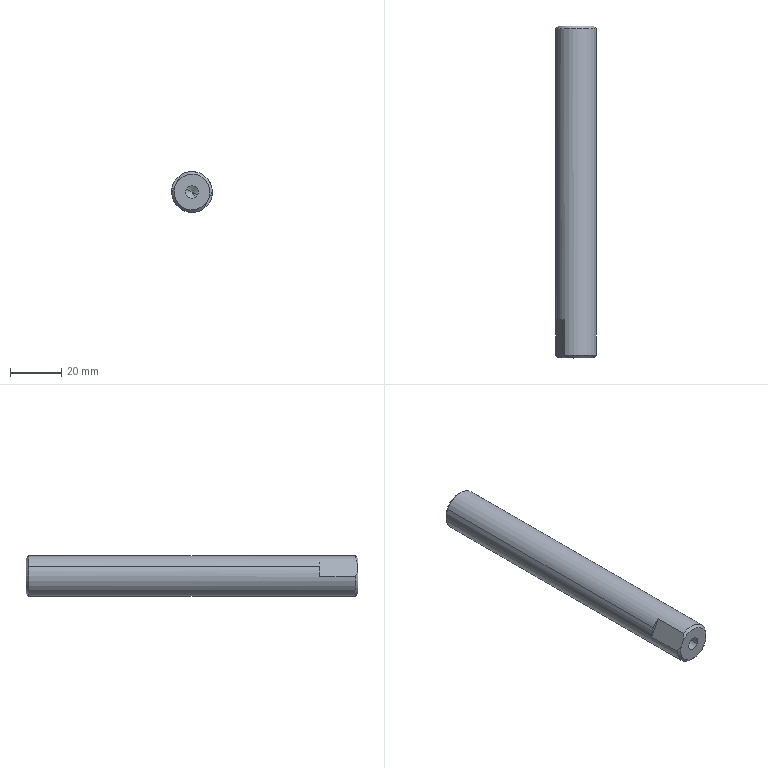Component | SolidWorks | PressingMechanism-25-2 | 1 solid | 16 faces | box 16 x 130 x 16 mm | volume 25596 mm3 | cone 6 | plane 6 | cylinder 4 | commonest cylinder face diameters 5 x2 16 x2
build123d program:
from build123d import *

# Parameters (mm, degrees)
SKETCH1_R             = 8
EXTRUDE1_DEPTH        = 130
M6_TAPPED_HOLE1_D     = 5
M6_TAPPED_HOLE1_DEPTH = 17
M6_TAPPED_HOLE1_TIP   = 1.502
CHAMFER1_SIZE         = 1
EXTRUDE2_DEPTH        = 131.491
EXTRUDE2_DEPTH_BACK   = 131.491
SKETCH4_W             = 15
SKETCH4_H             = 1


with BuildPart() as part:
    # Sketch1 → Extrude1 (new body)
    with BuildSketch(Plane(origin=(0, 0, 0), x_dir=(0, 0, -1), z_dir=(1, 0, 0))):
        Circle(SKETCH1_R)
    extrude(amount=EXTRUDE1_DEPTH)

    # M6 Tapped Hole1
    with Locations(Plane(origin=(130, 0, 0), x_dir=(0, 0, -1), z_dir=(1, 0, 0))):
        with Locations((0, 0)):
            Hole(M6_TAPPED_HOLE1_D / 2, depth=M6_TAPPED_HOLE1_DEPTH)
            with Locations((0, 0, -(M6_TAPPED_HOLE1_DEPTH + M6_TAPPED_HOLE1_TIP / 2))):  # 118° drill point
                Cone(0, M6_TAPPED_HOLE1_D / 2, M6_TAPPED_HOLE1_TIP, mode=Mode.SUBTRACT)

    # Chamfer1
    chamfer1_edges = [part.edges().sort_by_distance(p)[0] for p in [
        (0, 0, 8),
        (130, 0, 8),
    ]]
    chamfer(chamfer1_edges, length=CHAMFER1_SIZE)

    # Sketch4 → Extrude2 (cut, two sides: drawn at the far end of the back side and taken through both)
    with BuildSketch(Plane(origin=(0, 0, 0), x_dir=(1, 0, 0), z_dir=(0, 1, 0)).offset(-EXTRUDE2_DEPTH_BACK)):
        with Locations((122.5, 7.5)):
            Rectangle(SKETCH4_W, SKETCH4_H)
        with Locations((122.5, -7.5)):
            Rectangle(SKETCH4_W, SKETCH4_H)
    extrude(amount=EXTRUDE2_DEPTH + EXTRUDE2_DEPTH_BACK, mode=Mode.SUBTRACT)


solid = part.part

# Placed as in the assembly
solid = solid.moved(Location((0, -129, 61), (0, -62.719, -90)))
STEP:
#1=COLOUR_RGB('',0.7922,0.8196,0.9333);
#2=FILL_AREA_STYLE_COLOUR('',#1);
#3=FILL_AREA_STYLE('',(#2));
#4=SURFACE_STYLE_FILL_AREA(#3);
#5=SURFACE_SIDE_STYLE('',(#4));
#6=SURFACE_STYLE_USAGE(.BOTH.,#5);
#7=PRESENTATION_STYLE_ASSIGNMENT((#6));
#8=CARTESIAN_POINT('',(-0.2449,-5.079,2.528));
#9=VERTEX_POINT('',#8);
#10=CARTESIAN_POINT('',(0.2449,-5.079,2.275));
#11=VERTEX_POINT('',#10);
#12=CARTESIAN_POINT('',(0.,-5.079,2.402));
#13=DIRECTION('',(0.,1.,0.));
#14=DIRECTION('',(0.8888,0.,-0.4583));
#15=AXIS2_PLACEMENT_3D('',#12,#13,#14);
#16=CIRCLE('',#15,0.2756);
#17=EDGE_CURVE('',#9,#11,#16,.T.);
#18=ORIENTED_EDGE('',*,*,#17,.F.);
#19=CARTESIAN_POINT('',(-0.2799,-5.118,2.546));
#20=VERTEX_POINT('',#19);
#21=CARTESIAN_POINT('',(-0.2799,-5.118,2.546));
#22=DIRECTION('',(-0.6285,-0.7071,0.3241));
#23=VECTOR('',#22,39.37);
#24=LINE('',#21,#23);
#25=EDGE_CURVE('',#9,#20,#24,.T.);
#26=ORIENTED_EDGE('',*,*,#25,.T.);
#27=CARTESIAN_POINT('',(0.2799,-5.118,2.257));
#28=VERTEX_POINT('',#27);
#29=CARTESIAN_POINT('',(0.,-5.118,2.402));
#30=DIRECTION('',(0.,-1.,0.));
#31=DIRECTION('',(0.8888,0.,-0.4583));
#32=AXIS2_PLACEMENT_3D('',#29,#30,#31);
#33=CIRCLE('',#32,0.315);
#34=EDGE_CURVE('',#28,#20,#33,.T.);
#35=ORIENTED_EDGE('',*,*,#34,.F.);
#36=CARTESIAN_POINT('',(0.2799,-5.118,2.257));
#37=DIRECTION('',(0.6285,-0.7071,-0.3241));
#38=VECTOR('',#37,39.37);
#39=LINE('',#36,#38);
#40=EDGE_CURVE('',#11,#28,#39,.T.);
#41=ORIENTED_EDGE('',*,*,#40,.F.);
#42=EDGE_LOOP('',(#18,#26,#35,#41));
#43=FACE_OUTER_BOUND('',#42,.T.);
#44=CARTESIAN_POINT('',(0.,-5.118,2.402));
#45=DIRECTION('',(0.,-1.,0.));
#46=DIRECTION('',(0.8888,0.,-0.4583));
#47=AXIS2_PLACEMENT_3D('',#44,#45,#46);
#48=CONICAL_SURFACE('',#47,0.315,0.7854);
#49=ADVANCED_FACE('',(#43),#48,.T.);
#50=CARTESIAN_POINT('',(-0.08748,-9.528,2.447));
#51=VERTEX_POINT('',#50);
#52=CARTESIAN_POINT('',(0.08748,-9.528,2.356));
#53=VERTEX_POINT('',#52);
#54=CARTESIAN_POINT('',(0.,-9.528,2.402));
#55=DIRECTION('',(0.,-1.,0.));
#56=DIRECTION('',(0.8888,0.,-0.4583));
#57=AXIS2_PLACEMENT_3D('',#54,#55,#56);
#58=CIRCLE('',#57,0.09843);
#59=EDGE_CURVE('',#51,#53,#58,.T.);
#60=ORIENTED_EDGE('',*,*,#59,.F.);
#61=CARTESIAN_POINT('',(-0.08748,-10.197,2.447));
#62=VERTEX_POINT('',#61);
#63=CARTESIAN_POINT('',(-0.08748,-10.197,2.447));
#64=DIRECTION('',(0.,-1.,0.));
#65=VECTOR('',#64,39.37);
#66=LINE('',#63,#65);
#67=EDGE_CURVE('',#51,#62,#66,.T.);
#68=ORIENTED_EDGE('',*,*,#67,.T.);
#69=CARTESIAN_POINT('',(0.08748,-10.197,2.356));
#70=VERTEX_POINT('',#69);
#71=CARTESIAN_POINT('',(0.,-10.197,2.402));
#72=DIRECTION('',(0.,-1.,0.));
#73=DIRECTION('',(0.8888,0.,-0.4583));
#74=AXIS2_PLACEMENT_3D('',#71,#72,#73);
#75=CIRCLE('',#74,0.09843);
#76=EDGE_CURVE('',#62,#70,#75,.T.);
#77=ORIENTED_EDGE('',*,*,#76,.T.);
#78=CARTESIAN_POINT('',(0.08748,-10.197,2.356));
#79=DIRECTION('',(0.,-1.,0.));
#80=VECTOR('',#79,39.37);
#81=LINE('',#78,#80);
#82=EDGE_CURVE('',#53,#70,#81,.T.);
#83=ORIENTED_EDGE('',*,*,#82,.F.);
#84=EDGE_LOOP('',(#60,#68,#77,#83));
#85=FACE_OUTER_BOUND('',#84,.T.);
#86=CARTESIAN_POINT('',(0.,-10.197,2.402));
#87=DIRECTION('',(0.,-1.,0.));
#88=DIRECTION('',(0.8888,0.,-0.4583));
#89=AXIS2_PLACEMENT_3D('',#86,#87,#88);
#90=CYLINDRICAL_SURFACE('',#89,0.09843);
#91=ADVANCED_FACE('',(#85),#90,.F.);
#92=CARTESIAN_POINT('',(0.,-9.468,2.402));
#93=VERTEX_POINT('',#92);
#94=CARTESIAN_POINT('',(0.08748,-9.528,2.356));
#95=DIRECTION('',(0.7618,-0.515,-0.3929));
#96=VECTOR('',#95,39.37);
#97=LINE('',#94,#96);
#98=EDGE_CURVE('',#93,#53,#97,.T.);
#99=ORIENTED_EDGE('',*,*,#98,.F.);
#100=CARTESIAN_POINT('',(-0.08748,-9.528,2.447));
#101=DIRECTION('',(-0.7618,-0.515,0.3929));
#102=VECTOR('',#101,39.37);
#103=LINE('',#100,#102);
#104=EDGE_CURVE('',#93,#51,#103,.T.);
#105=ORIENTED_EDGE('',*,*,#104,.T.);
#106=ORIENTED_EDGE('',*,*,#59,.T.);
#107=EDGE_LOOP('',(#99,#105,#106));
#108=FACE_OUTER_BOUND('',#107,.T.);
#109=CARTESIAN_POINT('',(0.,-9.528,2.402));
#110=DIRECTION('',(0.,-1.,0.));
#111=DIRECTION('',(0.8888,0.,-0.4583));
#112=AXIS2_PLACEMENT_3D('',#109,#110,#111);
#113=CONICAL_SURFACE('',#112,0.09843,1.03);
#114=ADVANCED_FACE('',(#108),#113,.F.);
#115=CARTESIAN_POINT('',(0.3148,-9.606,2.411));
#116=VERTEX_POINT('',#115);
#117=CARTESIAN_POINT('',(0.2799,-9.606,2.257));
#118=VERTEX_POINT('',#117);
#119=CARTESIAN_POINT('',(0.,-9.606,2.402));
#120=DIRECTION('',(0.,1.,0.));
#121=DIRECTION('',(-0.8888,0.,0.4583));
#122=AXIS2_PLACEMENT_3D('',#119,#120,#121);
#123=CIRCLE('',#122,0.315);
#124=EDGE_CURVE('',#116,#118,#123,.T.);
#125=ORIENTED_EDGE('',*,*,#124,.T.);
#126=CARTESIAN_POINT('',(0.2799,-10.197,2.257));
#127=DIRECTION('',(0.,1.,0.));
#128=VECTOR('',#127,39.37);
#129=LINE('',#126,#128);
#130=EDGE_CURVE('',#118,#28,#129,.T.);
#131=ORIENTED_EDGE('',*,*,#130,.T.);
#132=ORIENTED_EDGE('',*,*,#34,.T.);
#133=CARTESIAN_POINT('',(-0.2799,-9.606,2.546));
#134=VERTEX_POINT('',#133);
#135=CARTESIAN_POINT('',(-0.2799,-10.197,2.546));
#136=DIRECTION('',(0.,1.,0.));
#137=VECTOR('',#136,39.37);
#138=LINE('',#135,#137);
#139=EDGE_CURVE('',#134,#20,#138,.T.);
#140=ORIENTED_EDGE('',*,*,#139,.F.);
#141=CARTESIAN_POINT('',(-0.1751,-9.606,2.663));
#142=VERTEX_POINT('',#141);
#143=CARTESIAN_POINT('',(0.,-9.606,2.402));
#144=DIRECTION('',(0.,1.,0.));
#145=DIRECTION('',(-0.8888,0.,0.4583));
#146=AXIS2_PLACEMENT_3D('',#143,#144,#145);
#147=CIRCLE('',#146,0.315);
#148=EDGE_CURVE('',#134,#142,#147,.T.);
#149=ORIENTED_EDGE('',*,*,#148,.T.);
#150=CARTESIAN_POINT('',(-0.1751,-10.157,2.663));
#151=VERTEX_POINT('',#150);
#152=CARTESIAN_POINT('',(-0.1751,-10.197,2.663));
#153=DIRECTION('',(0.,-1.,0.));
#154=VECTOR('',#153,39.37);
#155=LINE('',#152,#154);
#156=EDGE_CURVE('',#142,#151,#155,.T.);
#157=ORIENTED_EDGE('',*,*,#156,.T.);
#158=CARTESIAN_POINT('',(0.3148,-10.157,2.411));
#159=VERTEX_POINT('',#158);
#160=CARTESIAN_POINT('',(0.,-10.157,2.402));
#161=DIRECTION('',(0.,1.,0.));
#162=DIRECTION('',(0.8888,0.,-0.4583));
#163=AXIS2_PLACEMENT_3D('',#160,#161,#162);
#164=CIRCLE('',#163,0.315);
#165=EDGE_CURVE('',#151,#159,#164,.T.);
#166=ORIENTED_EDGE('',*,*,#165,.T.);
#167=CARTESIAN_POINT('',(0.3148,-10.197,2.411));
#168=DIRECTION('',(0.,1.,0.));
#169=VECTOR('',#168,39.37);
#170=LINE('',#167,#169);
#171=EDGE_CURVE('',#159,#116,#170,.T.);
#172=ORIENTED_EDGE('',*,*,#171,.T.);
#173=EDGE_LOOP('',(#125,#131,#132,#140,#149,#157,#166,#172));
#174=FACE_OUTER_BOUND('',#173,.T.);
#175=CARTESIAN_POINT('',(0.,-10.197,2.402));
#176=DIRECTION('',(0.,1.,0.));
#177=DIRECTION('',(-0.8888,0.,0.4583));
#178=AXIS2_PLACEMENT_3D('',#175,#176,#177);
#179=CYLINDRICAL_SURFACE('',#178,0.315);
#180=ADVANCED_FACE('',(#174),#179,.T.);
#181=CARTESIAN_POINT('',(-0.3148,-10.157,2.392));
#182=VERTEX_POINT('',#181);
#183=CARTESIAN_POINT('',(-0.2449,-10.197,2.528));
#184=VERTEX_POINT('',#183);
#185=CARTESIAN_POINT('',(-0.3148,-10.157,2.392));
#186=CARTESIAN_POINT('',(-0.3041,-10.169,2.413));
#187=CARTESIAN_POINT('',(-0.2929,-10.179,2.435));
#188=CARTESIAN_POINT('',(-0.2692,-10.193,2.481));
#189=CARTESIAN_POINT('',(-0.2572,-10.197,2.504));
#190=CARTESIAN_POINT('',(-0.2449,-10.197,2.528));
#191=B_SPLINE_CURVE_WITH_KNOTS('',3,(#185,#186,#187,#188,#189,#190),.UNSPECIFIED.,.F.,.F.,(4,2,4),(0.02013,0.02213,0.02413),.UNSPECIFIED.);
#192=EDGE_CURVE('',#182,#184,#191,.T.);
#193=ORIENTED_EDGE('',*,*,#192,.F.);
#194=CARTESIAN_POINT('',(0.1751,-10.157,2.14));
#195=VERTEX_POINT('',#194);
#196=CARTESIAN_POINT('',(0.,-10.157,2.402));
#197=DIRECTION('',(0.,1.,0.));
#198=DIRECTION('',(0.8888,0.,-0.4583));
#199=AXIS2_PLACEMENT_3D('',#196,#197,#198);
#200=CIRCLE('',#199,0.315);
#201=EDGE_CURVE('',#195,#182,#200,.T.);
#202=ORIENTED_EDGE('',*,*,#201,.F.);
#203=CARTESIAN_POINT('',(0.2449,-10.197,2.275));
#204=VERTEX_POINT('',#203);
#205=CARTESIAN_POINT('',(0.2449,-10.197,2.275));
#206=CARTESIAN_POINT('',(0.2327,-10.197,2.251));
#207=CARTESIAN_POINT('',(0.2206,-10.193,2.228));
#208=CARTESIAN_POINT('',(0.197,-10.179,2.182));
#209=CARTESIAN_POINT('',(0.1858,-10.169,2.161));
#210=CARTESIAN_POINT('',(0.1751,-10.157,2.14));
#211=B_SPLINE_CURVE_WITH_KNOTS('',3,(#205,#206,#207,#208,#209,#210),.UNSPECIFIED.,.F.,.F.,(4,2,4),(0.008364,0.01037,0.01237),.UNSPECIFIED.);
#212=EDGE_CURVE('',#204,#195,#211,.T.);
#213=ORIENTED_EDGE('',*,*,#212,.F.);
#214=CARTESIAN_POINT('',(0.,-10.197,2.402));
#215=DIRECTION('',(0.,-1.,0.));
#216=DIRECTION('',(0.8888,0.,-0.4583));
#217=AXIS2_PLACEMENT_3D('',#214,#215,#216);
#218=CIRCLE('',#217,0.2756);
#219=EDGE_CURVE('',#184,#204,#218,.T.);
#220=ORIENTED_EDGE('',*,*,#219,.F.);
#221=EDGE_LOOP('',(#193,#202,#213,#220));
#222=FACE_OUTER_BOUND('',#221,.T.);
#223=CARTESIAN_POINT('',(0.,-10.197,2.402));
#224=DIRECTION('',(0.,1.,0.));
#225=DIRECTION('',(-0.8888,0.,0.4583));
#226=AXIS2_PLACEMENT_3D('',#223,#224,#225);
#227=CONICAL_SURFACE('',#226,0.2756,0.7854);
#228=ADVANCED_FACE('',(#222),#227,.T.);
#229=ORIENTED_EDGE('',*,*,#130,.F.);
#230=CARTESIAN_POINT('',(0.1751,-9.606,2.14));
#231=VERTEX_POINT('',#230);
#232=CARTESIAN_POINT('',(0.,-9.606,2.402));
#233=DIRECTION('',(0.,1.,0.));
#234=DIRECTION('',(-0.8888,0.,0.4583));
#235=AXIS2_PLACEMENT_3D('',#232,#233,#234);
#236=CIRCLE('',#235,0.315);
#237=EDGE_CURVE('',#118,#231,#236,.T.);
#238=ORIENTED_EDGE('',*,*,#237,.T.);
#239=CARTESIAN_POINT('',(0.1751,-10.197,2.14));
#240=DIRECTION('',(0.,-1.,0.));
#241=VECTOR('',#240,39.37);
#242=LINE('',#239,#241);
#243=EDGE_CURVE('',#231,#195,#242,.T.);
#244=ORIENTED_EDGE('',*,*,#243,.T.);
#245=ORIENTED_EDGE('',*,*,#201,.T.);
#246=CARTESIAN_POINT('',(-0.3148,-9.606,2.392));
#247=VERTEX_POINT('',#246);
#248=CARTESIAN_POINT('',(-0.3148,-10.197,2.392));
#249=DIRECTION('',(0.,1.,0.));
#250=VECTOR('',#249,39.37);
#251=LINE('',#248,#250);
#252=EDGE_CURVE('',#182,#247,#251,.T.);
#253=ORIENTED_EDGE('',*,*,#252,.T.);
#254=CARTESIAN_POINT('',(0.,-9.606,2.402));
#255=DIRECTION('',(0.,1.,0.));
#256=DIRECTION('',(-0.8888,0.,0.4583));
#257=AXIS2_PLACEMENT_3D('',#254,#255,#256);
#258=CIRCLE('',#257,0.315);
#259=EDGE_CURVE('',#247,#134,#258,.T.);
#260=ORIENTED_EDGE('',*,*,#259,.T.);
#261=ORIENTED_EDGE('',*,*,#139,.T.);
#262=CARTESIAN_POINT('',(0.,-5.118,2.402));
#263=DIRECTION('',(0.,-1.,0.));
#264=DIRECTION('',(0.8888,0.,-0.4583));
#265=AXIS2_PLACEMENT_3D('',#262,#263,#264);
#266=CIRCLE('',#265,0.315);
#267=EDGE_CURVE('',#20,#28,#266,.T.);
#268=ORIENTED_EDGE('',*,*,#267,.T.);
#269=EDGE_LOOP('',(#229,#238,#244,#245,#253,#260,#261,#268));
#270=FACE_OUTER_BOUND('',#269,.T.);
#271=CARTESIAN_POINT('',(0.,-10.197,2.402));
#272=DIRECTION('',(0.,1.,0.));
#273=DIRECTION('',(-0.8888,0.,0.4583));
#274=AXIS2_PLACEMENT_3D('',#271,#272,#273);
#275=CYLINDRICAL_SURFACE('',#274,0.315);
#276=ADVANCED_FACE('',(#270),#275,.T.);
#277=CARTESIAN_POINT('',(0.,-10.197,2.402));
#278=DIRECTION('',(0.,-1.,0.));
#279=DIRECTION('',(0.8888,0.,-0.4583));
#280=AXIS2_PLACEMENT_3D('',#277,#278,#279);
#281=CIRCLE('',#280,0.2756);
#282=EDGE_CURVE('',#204,#184,#281,.T.);
#283=ORIENTED_EDGE('',*,*,#282,.T.);
#284=ORIENTED_EDGE('',*,*,#219,.T.);
#285=EDGE_LOOP('',(#283,#284));
#286=FACE_OUTER_BOUND('',#285,.T.);
#287=CARTESIAN_POINT('',(0.,-10.197,2.402));
#288=DIRECTION('',(0.,-1.,0.));
#289=DIRECTION('',(0.8888,0.,-0.4583));
#290=AXIS2_PLACEMENT_3D('',#287,#288,#289);
#291=CIRCLE('',#290,0.09843);
#292=EDGE_CURVE('',#70,#62,#291,.T.);
#293=ORIENTED_EDGE('',*,*,#292,.F.);
#294=ORIENTED_EDGE('',*,*,#76,.F.);
#295=EDGE_LOOP('',(#293,#294));
#296=FACE_BOUND('',#295,.T.);
#297=CARTESIAN_POINT('',(0.,-10.197,2.402));
#298=DIRECTION('',(0.,-1.,0.));
#299=DIRECTION('',(0.8888,0.,-0.4583));
#300=AXIS2_PLACEMENT_3D('',#297,#298,#299);
#301=PLANE('',#300);
#302=ADVANCED_FACE('',(#286,#296),#301,.T.);
#303=CARTESIAN_POINT('',(0.,-5.079,2.402));
#304=DIRECTION('',(0.,1.,0.));
#305=DIRECTION('',(0.8888,0.,-0.4583));
#306=AXIS2_PLACEMENT_3D('',#303,#304,#305);
#307=CIRCLE('',#306,0.2756);
#308=EDGE_CURVE('',#11,#9,#307,.T.);
#309=ORIENTED_EDGE('',*,*,#308,.T.);
#310=ORIENTED_EDGE('',*,*,#17,.T.);
#311=EDGE_LOOP('',(#309,#310));
#312=FACE_OUTER_BOUND('',#311,.T.);
#313=CARTESIAN_POINT('',(0.,-5.079,2.402));
#314=DIRECTION('',(0.,-1.,0.));
#315=DIRECTION('',(0.8888,0.,-0.4583));
#316=AXIS2_PLACEMENT_3D('',#313,#314,#315);
#317=PLANE('',#316);
#318=ADVANCED_FACE('',(#312),#317,.F.);
#319=ORIENTED_EDGE('',*,*,#104,.F.);
#320=ORIENTED_EDGE('',*,*,#98,.T.);
#321=CARTESIAN_POINT('',(0.,-9.528,2.402));
#322=DIRECTION('',(0.,-1.,0.));
#323=DIRECTION('',(0.8888,0.,-0.4583));
#324=AXIS2_PLACEMENT_3D('',#321,#322,#323);
#325=CIRCLE('',#324,0.09843);
#326=EDGE_CURVE('',#53,#51,#325,.T.);
#327=ORIENTED_EDGE('',*,*,#326,.T.);
#328=EDGE_LOOP('',(#319,#320,#327));
#329=FACE_OUTER_BOUND('',#328,.T.);
#330=CARTESIAN_POINT('',(0.,-9.528,2.402));
#331=DIRECTION('',(0.,-1.,0.));
#332=DIRECTION('',(0.8888,0.,-0.4583));
#333=AXIS2_PLACEMENT_3D('',#330,#331,#332);
#334=CONICAL_SURFACE('',#333,0.09843,1.03);
#335=ADVANCED_FACE('',(#329),#334,.F.);
#336=ORIENTED_EDGE('',*,*,#67,.F.);
#337=ORIENTED_EDGE('',*,*,#326,.F.);
#338=ORIENTED_EDGE('',*,*,#82,.T.);
#339=ORIENTED_EDGE('',*,*,#292,.T.);
#340=EDGE_LOOP('',(#336,#337,#338,#339));
#341=FACE_OUTER_BOUND('',#340,.T.);
#342=CARTESIAN_POINT('',(0.,-10.197,2.402));
#343=DIRECTION('',(0.,-1.,0.));
#344=DIRECTION('',(0.8888,0.,-0.4583));
#345=AXIS2_PLACEMENT_3D('',#342,#343,#344);
#346=CYLINDRICAL_SURFACE('',#345,0.09843);
#347=ADVANCED_FACE('',(#341),#346,.F.);
#348=ORIENTED_EDGE('',*,*,#25,.F.);
#349=ORIENTED_EDGE('',*,*,#308,.F.);
#350=ORIENTED_EDGE('',*,*,#40,.T.);
#351=ORIENTED_EDGE('',*,*,#267,.F.);
#352=EDGE_LOOP('',(#348,#349,#350,#351));
#353=FACE_OUTER_BOUND('',#352,.T.);
#354=CARTESIAN_POINT('',(0.,-5.118,2.402));
#355=DIRECTION('',(0.,-1.,0.));
#356=DIRECTION('',(0.8888,0.,-0.4583));
#357=AXIS2_PLACEMENT_3D('',#354,#355,#356);
#358=CONICAL_SURFACE('',#357,0.315,0.7854);
#359=ADVANCED_FACE('',(#353),#358,.T.);
#360=CARTESIAN_POINT('',(-0.2449,-10.197,2.528));
#361=CARTESIAN_POINT('',(-0.2388,-10.197,2.54));
#362=CARTESIAN_POINT('',(-0.2327,-10.196,2.552));
#363=CARTESIAN_POINT('',(-0.2208,-10.192,2.575));
#364=CARTESIAN_POINT('',(-0.2148,-10.189,2.586));
#365=CARTESIAN_POINT('',(-0.2031,-10.182,2.609));
#366=CARTESIAN_POINT('',(-0.1973,-10.178,2.62));
#367=CARTESIAN_POINT('',(-0.186,-10.169,2.642));
#368=CARTESIAN_POINT('',(-0.1805,-10.163,2.653));
#369=CARTESIAN_POINT('',(-0.1751,-10.157,2.663));
#370=B_SPLINE_CURVE_WITH_KNOTS('',3,(#360,#361,#362,#363,#364,#365,#366,#367,#368,#369),.UNSPECIFIED.,.F.,.F.,(4,2,2,2,4),(0.02413,0.02513,0.02612,0.02712,0.02812),.UNSPECIFIED.);
#371=EDGE_CURVE('',#184,#151,#370,.T.);
#372=ORIENTED_EDGE('',*,*,#371,.F.);
#373=ORIENTED_EDGE('',*,*,#282,.F.);
#374=CARTESIAN_POINT('',(0.3148,-10.157,2.411));
#375=CARTESIAN_POINT('',(0.3094,-10.163,2.4));
#376=CARTESIAN_POINT('',(0.3039,-10.169,2.39));
#377=CARTESIAN_POINT('',(0.2926,-10.178,2.368));
#378=CARTESIAN_POINT('',(0.2867,-10.182,2.356));
#379=CARTESIAN_POINT('',(0.275,-10.189,2.334));
#380=CARTESIAN_POINT('',(0.2691,-10.192,2.322));
#381=CARTESIAN_POINT('',(0.2571,-10.196,2.299));
#382=CARTESIAN_POINT('',(0.2511,-10.197,2.287));
#383=CARTESIAN_POINT('',(0.2449,-10.197,2.275));
#384=B_SPLINE_CURVE_WITH_KNOTS('',3,(#374,#375,#376,#377,#378,#379,#380,#381,#382,#383),.UNSPECIFIED.,.F.,.F.,(4,2,2,2,4),(0.004369,0.005367,0.006366,0.007365,0.008364),.UNSPECIFIED.);
#385=EDGE_CURVE('',#159,#204,#384,.T.);
#386=ORIENTED_EDGE('',*,*,#385,.F.);
#387=ORIENTED_EDGE('',*,*,#165,.F.);
#388=EDGE_LOOP('',(#372,#373,#386,#387));
#389=FACE_OUTER_BOUND('',#388,.T.);
#390=CARTESIAN_POINT('',(0.,-10.197,2.402));
#391=DIRECTION('',(0.,1.,0.));
#392=DIRECTION('',(-0.8888,0.,0.4583));
#393=AXIS2_PLACEMENT_3D('',#390,#391,#392);
#394=CONICAL_SURFACE('',#393,0.2756,0.7854);
#395=ADVANCED_FACE('',(#389),#394,.T.);
#396=CARTESIAN_POINT('',(0.1006,-9.606,1.995));
#397=DIRECTION('',(0.4583,0.,0.8888));
#398=VECTOR('',#397,39.37);
#399=LINE('',#396,#398);
#400=EDGE_CURVE('',#231,#116,#399,.T.);
#401=ORIENTED_EDGE('',*,*,#400,.F.);
#402=ORIENTED_EDGE('',*,*,#237,.F.);
#403=ORIENTED_EDGE('',*,*,#124,.F.);
#404=EDGE_LOOP('',(#401,#402,#403));
#405=FACE_OUTER_BOUND('',#404,.T.);
#406=CARTESIAN_POINT('',(0.1356,-9.606,1.977));
#407=DIRECTION('',(0.,1.,0.));
#408=DIRECTION('',(-0.8888,0.,0.4583));
#409=AXIS2_PLACEMENT_3D('',#406,#407,#408);
#410=PLANE('',#409);
#411=ADVANCED_FACE('',(#405),#410,.F.);
#412=ORIENTED_EDGE('',*,*,#385,.T.);
#413=ORIENTED_EDGE('',*,*,#212,.T.);
#414=ORIENTED_EDGE('',*,*,#243,.F.);
#415=ORIENTED_EDGE('',*,*,#400,.T.);
#416=ORIENTED_EDGE('',*,*,#171,.F.);
#417=EDGE_LOOP('',(#412,#413,#414,#415,#416));
#418=FACE_OUTER_BOUND('',#417,.T.);
#419=CARTESIAN_POINT('',(0.1006,-10.197,1.995));
#420=DIRECTION('',(-0.8888,-0.,0.4583));
#421=DIRECTION('',(0.,-1.,-0.));
#422=AXIS2_PLACEMENT_3D('',#419,#420,#421);
#423=PLANE('',#422);
#424=ADVANCED_FACE('',(#418),#423,.F.);
#425=ORIENTED_EDGE('',*,*,#259,.F.);
#426=CARTESIAN_POINT('',(-0.3893,-9.606,2.248));
#427=DIRECTION('',(0.4583,0.,0.8888));
#428=VECTOR('',#427,39.37);
#429=LINE('',#426,#428);
#430=EDGE_CURVE('',#247,#142,#429,.T.);
#431=ORIENTED_EDGE('',*,*,#430,.T.);
#432=ORIENTED_EDGE('',*,*,#148,.F.);
#433=EDGE_LOOP('',(#425,#431,#432));
#434=FACE_OUTER_BOUND('',#433,.T.);
#435=CARTESIAN_POINT('',(-0.4243,-9.606,2.266));
#436=DIRECTION('',(0.,1.,0.));
#437=DIRECTION('',(-0.8888,0.,0.4583));
#438=AXIS2_PLACEMENT_3D('',#435,#436,#437);
#439=PLANE('',#438);
#440=ADVANCED_FACE('',(#434),#439,.F.);
#441=ORIENTED_EDGE('',*,*,#192,.T.);
#442=ORIENTED_EDGE('',*,*,#371,.T.);
#443=ORIENTED_EDGE('',*,*,#156,.F.);
#444=ORIENTED_EDGE('',*,*,#430,.F.);
#445=ORIENTED_EDGE('',*,*,#252,.F.);
#446=EDGE_LOOP('',(#441,#442,#443,#444,#445));
#447=FACE_OUTER_BOUND('',#446,.T.);
#448=CARTESIAN_POINT('',(-0.3893,-10.197,2.248));
#449=DIRECTION('',(0.8888,-0.,-0.4583));
#450=DIRECTION('',(0.,1.,-0.));
#451=AXIS2_PLACEMENT_3D('',#448,#449,#450);
#452=PLANE('',#451);
#453=ADVANCED_FACE('',(#447),#452,.F.);
#454=CLOSED_SHELL('',(#49,#91,#114,#180,#228,#276,#302,#318,#335,#347,#359,#395,#411,#424,#440,#453));
#455=MANIFOLD_SOLID_BREP('',#454);
#456=STYLED_ITEM('',(#7),#455);
#457=PRESENTATION_LAYER_ASSIGNMENT('','',(#456));
#458=CARTESIAN_POINT('',(0.,0.,0.));
#459=DIRECTION('',(0.,0.,1.));
#460=DIRECTION('',(1.,0.,0.));
#461=AXIS2_PLACEMENT_3D('',#458,#459,#460);
#462=(LENGTH_UNIT()NAMED_UNIT(*)SI_UNIT($,.METRE.));
#463=LENGTH_MEASURE_WITH_UNIT(LENGTH_MEASURE(0.0254),#462);
#464=DIMENSIONAL_EXPONENTS(1.,0.,0.,0.,0.,0.,0.);
#465=(CONVERSION_BASED_UNIT('',#463)LENGTH_UNIT()NAMED_UNIT(#464));
#466=UNCERTAINTY_MEASURE_WITH_UNIT(LENGTH_MEASURE(0.00001),#465,'','');
#467=(NAMED_UNIT(*)PLANE_ANGLE_UNIT()SI_UNIT($,.RADIAN.));
#468=(NAMED_UNIT(*)SI_UNIT($,.STERADIAN.)SOLID_ANGLE_UNIT());
#469=(GEOMETRIC_REPRESENTATION_CONTEXT(3)GLOBAL_UNCERTAINTY_ASSIGNED_CONTEXT((#466))GLOBAL_UNIT_ASSIGNED_CONTEXT((#465,#467,#468))REPRESENTATION_CONTEXT('',''));
#470=ADVANCED_BREP_SHAPE_REPRESENTATION('',(#455,#461),#469);
#471=(LENGTH_UNIT()NAMED_UNIT(*)SI_UNIT($,.METRE.));
#472=LENGTH_MEASURE_WITH_UNIT(LENGTH_MEASURE(0.0254),#471);
#473=DIMENSIONAL_EXPONENTS(1.,0.,0.,0.,0.,0.,0.);
#474=(CONVERSION_BASED_UNIT('',#472)LENGTH_UNIT()NAMED_UNIT(#473));
#475=UNCERTAINTY_MEASURE_WITH_UNIT(LENGTH_MEASURE(0.00001),#474,'','');
#476=(NAMED_UNIT(*)PLANE_ANGLE_UNIT()SI_UNIT($,.RADIAN.));
#477=(NAMED_UNIT(*)SI_UNIT($,.STERADIAN.)SOLID_ANGLE_UNIT());
#478=(GEOMETRIC_REPRESENTATION_CONTEXT(3)GLOBAL_UNCERTAINTY_ASSIGNED_CONTEXT((#475))GLOBAL_UNIT_ASSIGNED_CONTEXT((#474,#476,#477))REPRESENTATION_CONTEXT('',''));
#479=MECHANICAL_DESIGN_GEOMETRIC_PRESENTATION_REPRESENTATION('',(#456),#478);